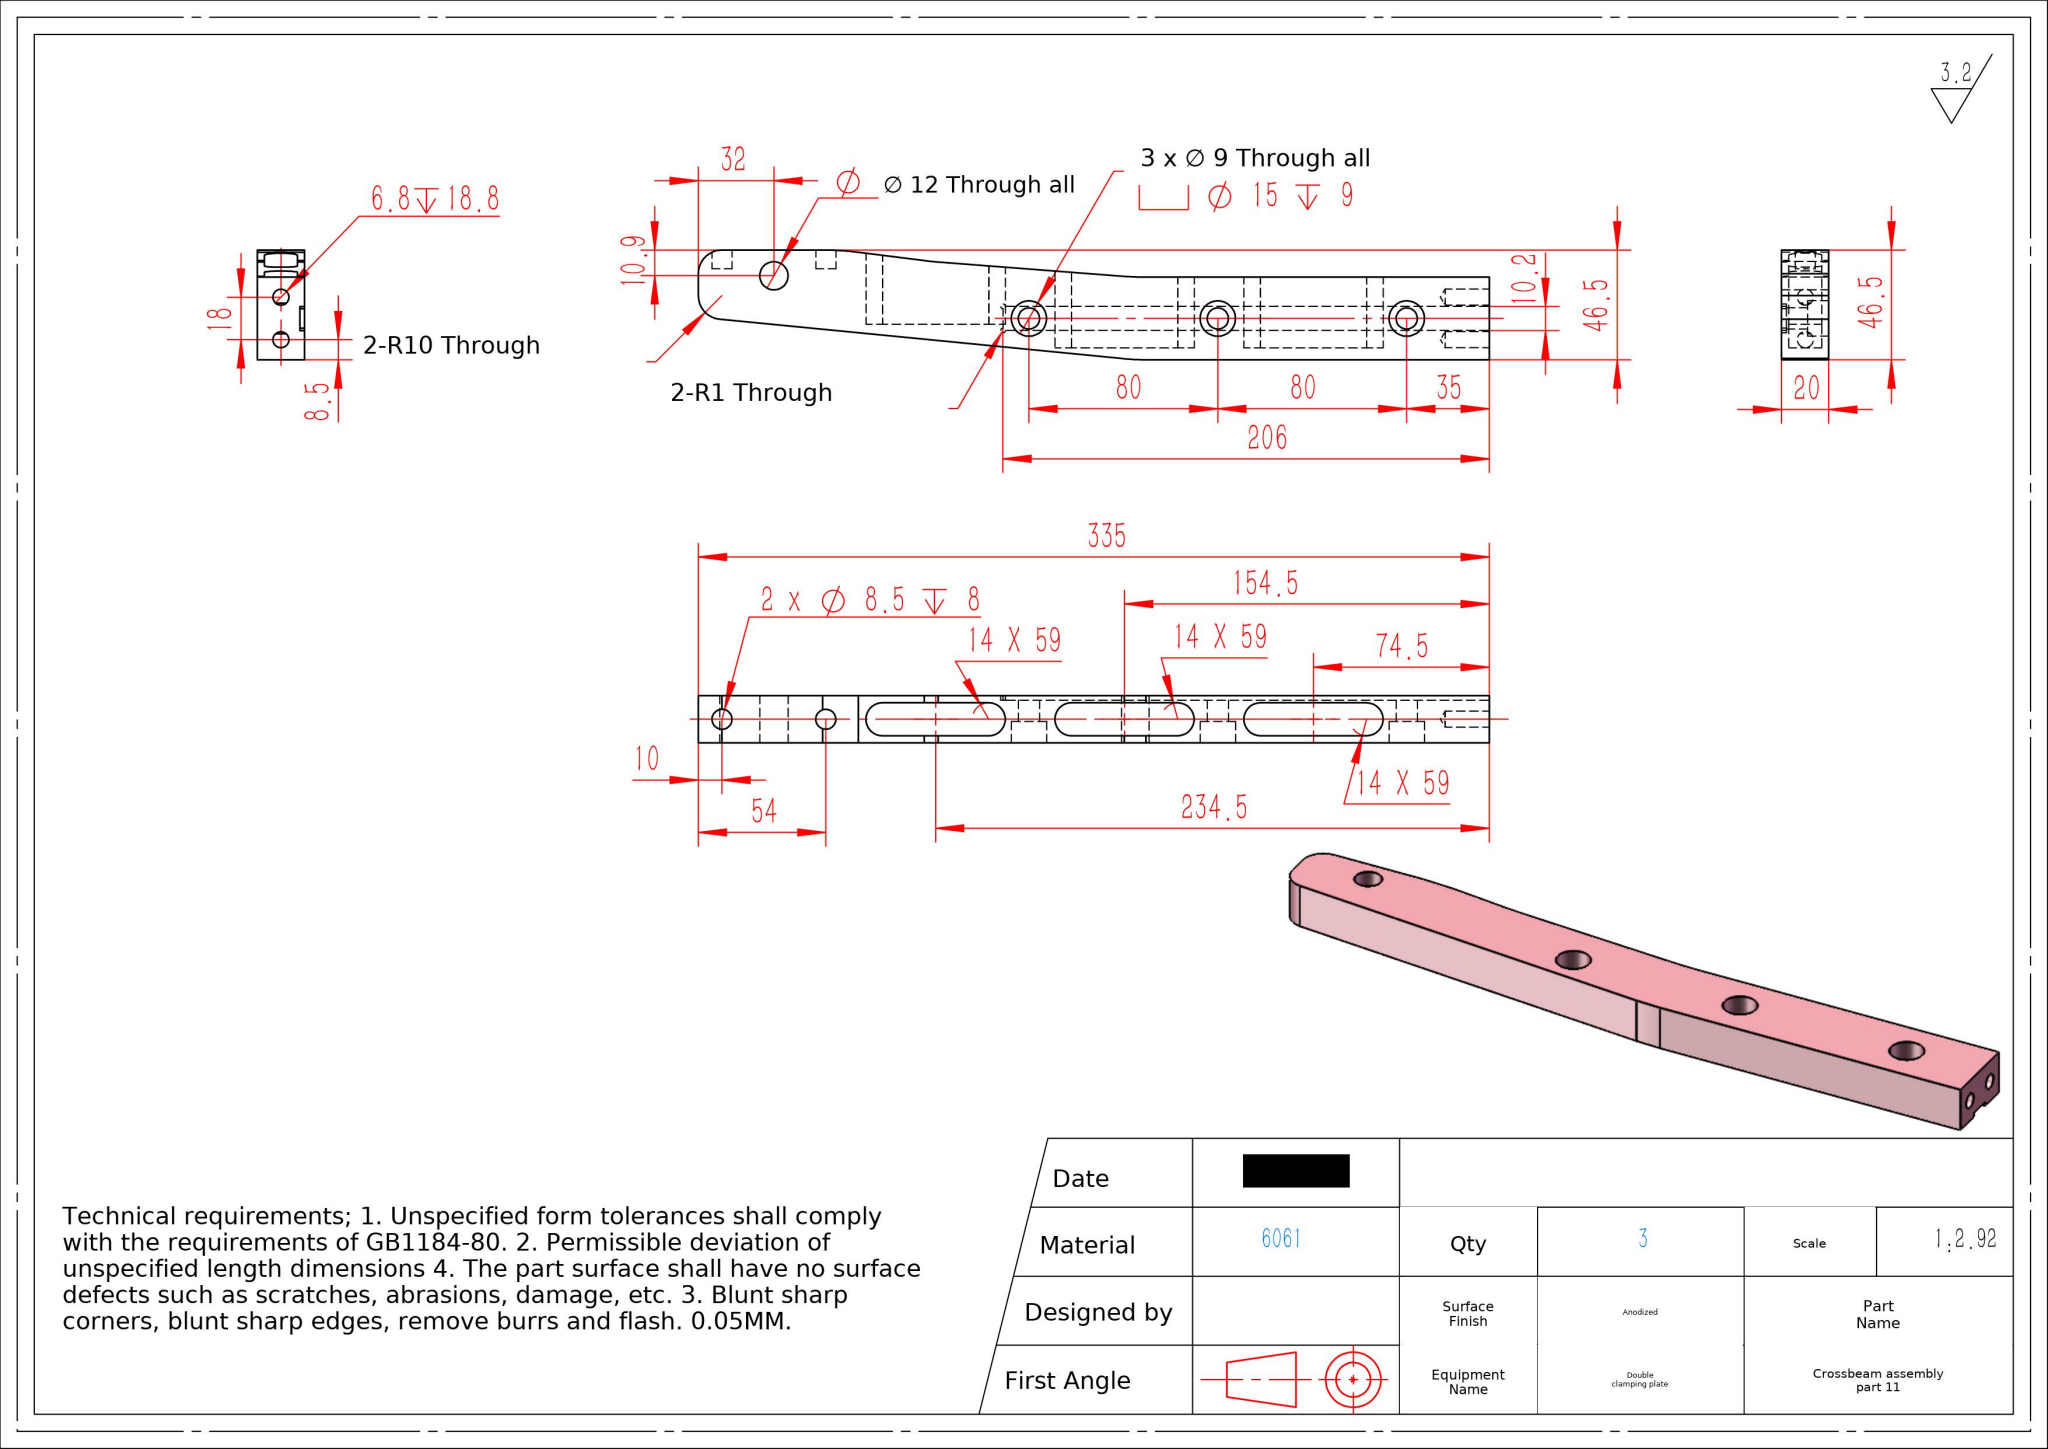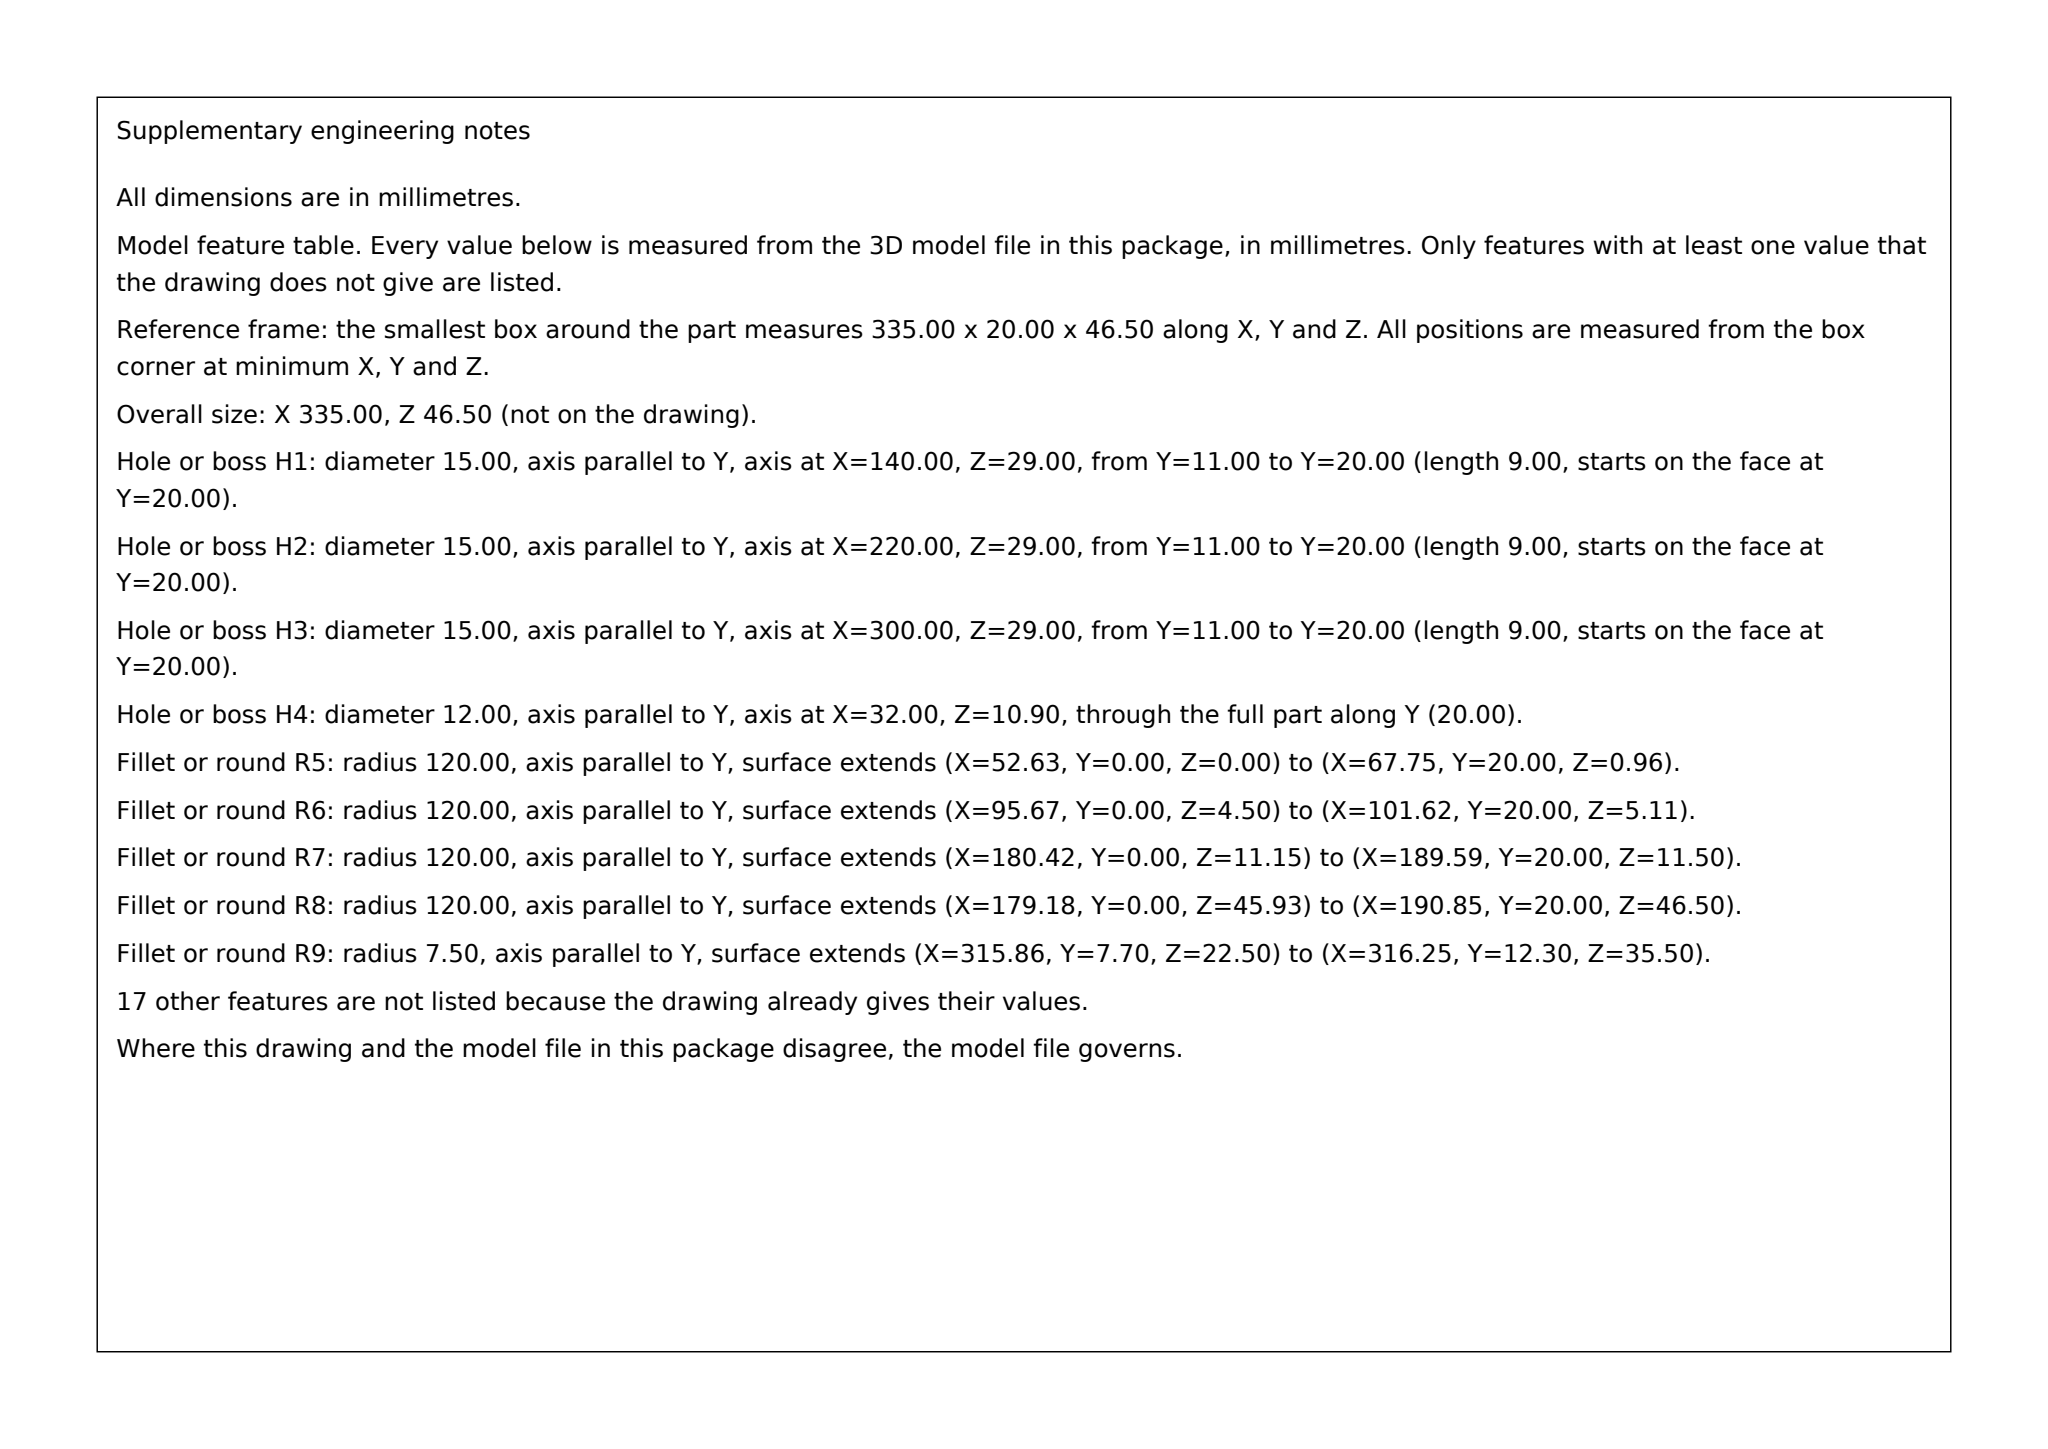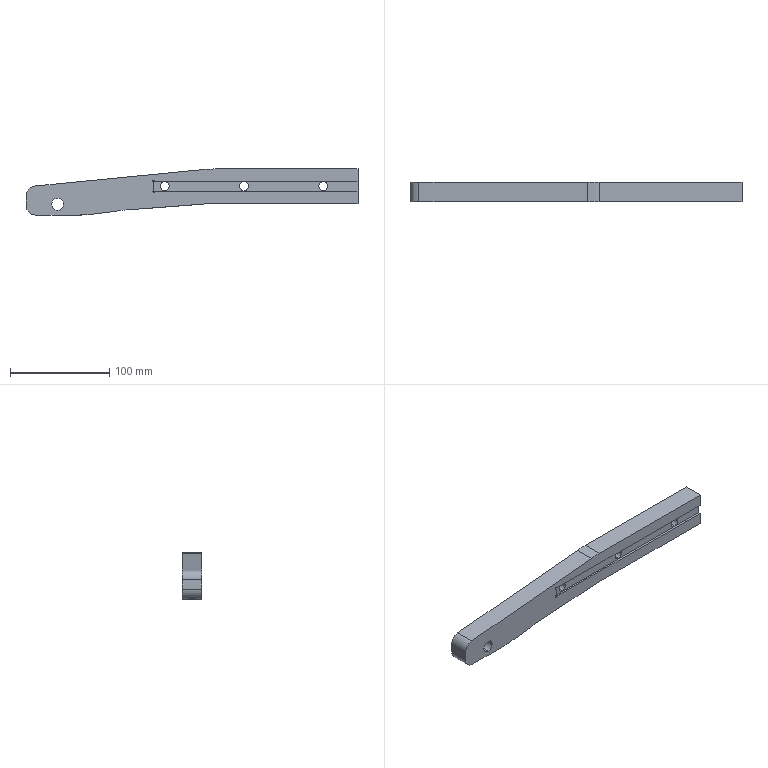Part | SolidWorks | mm | material 6061 | 1 solid | 78 faces | box 335 x 20 x 46.5 mm | volume 142904 mm3 | cylinder 44 | plane 30 | cone 4 | commonest cylinder face diameters 14 x9 15 x8 9 x6 240 x6 8.5 x4 6.8 x4 2 x3 12 x2